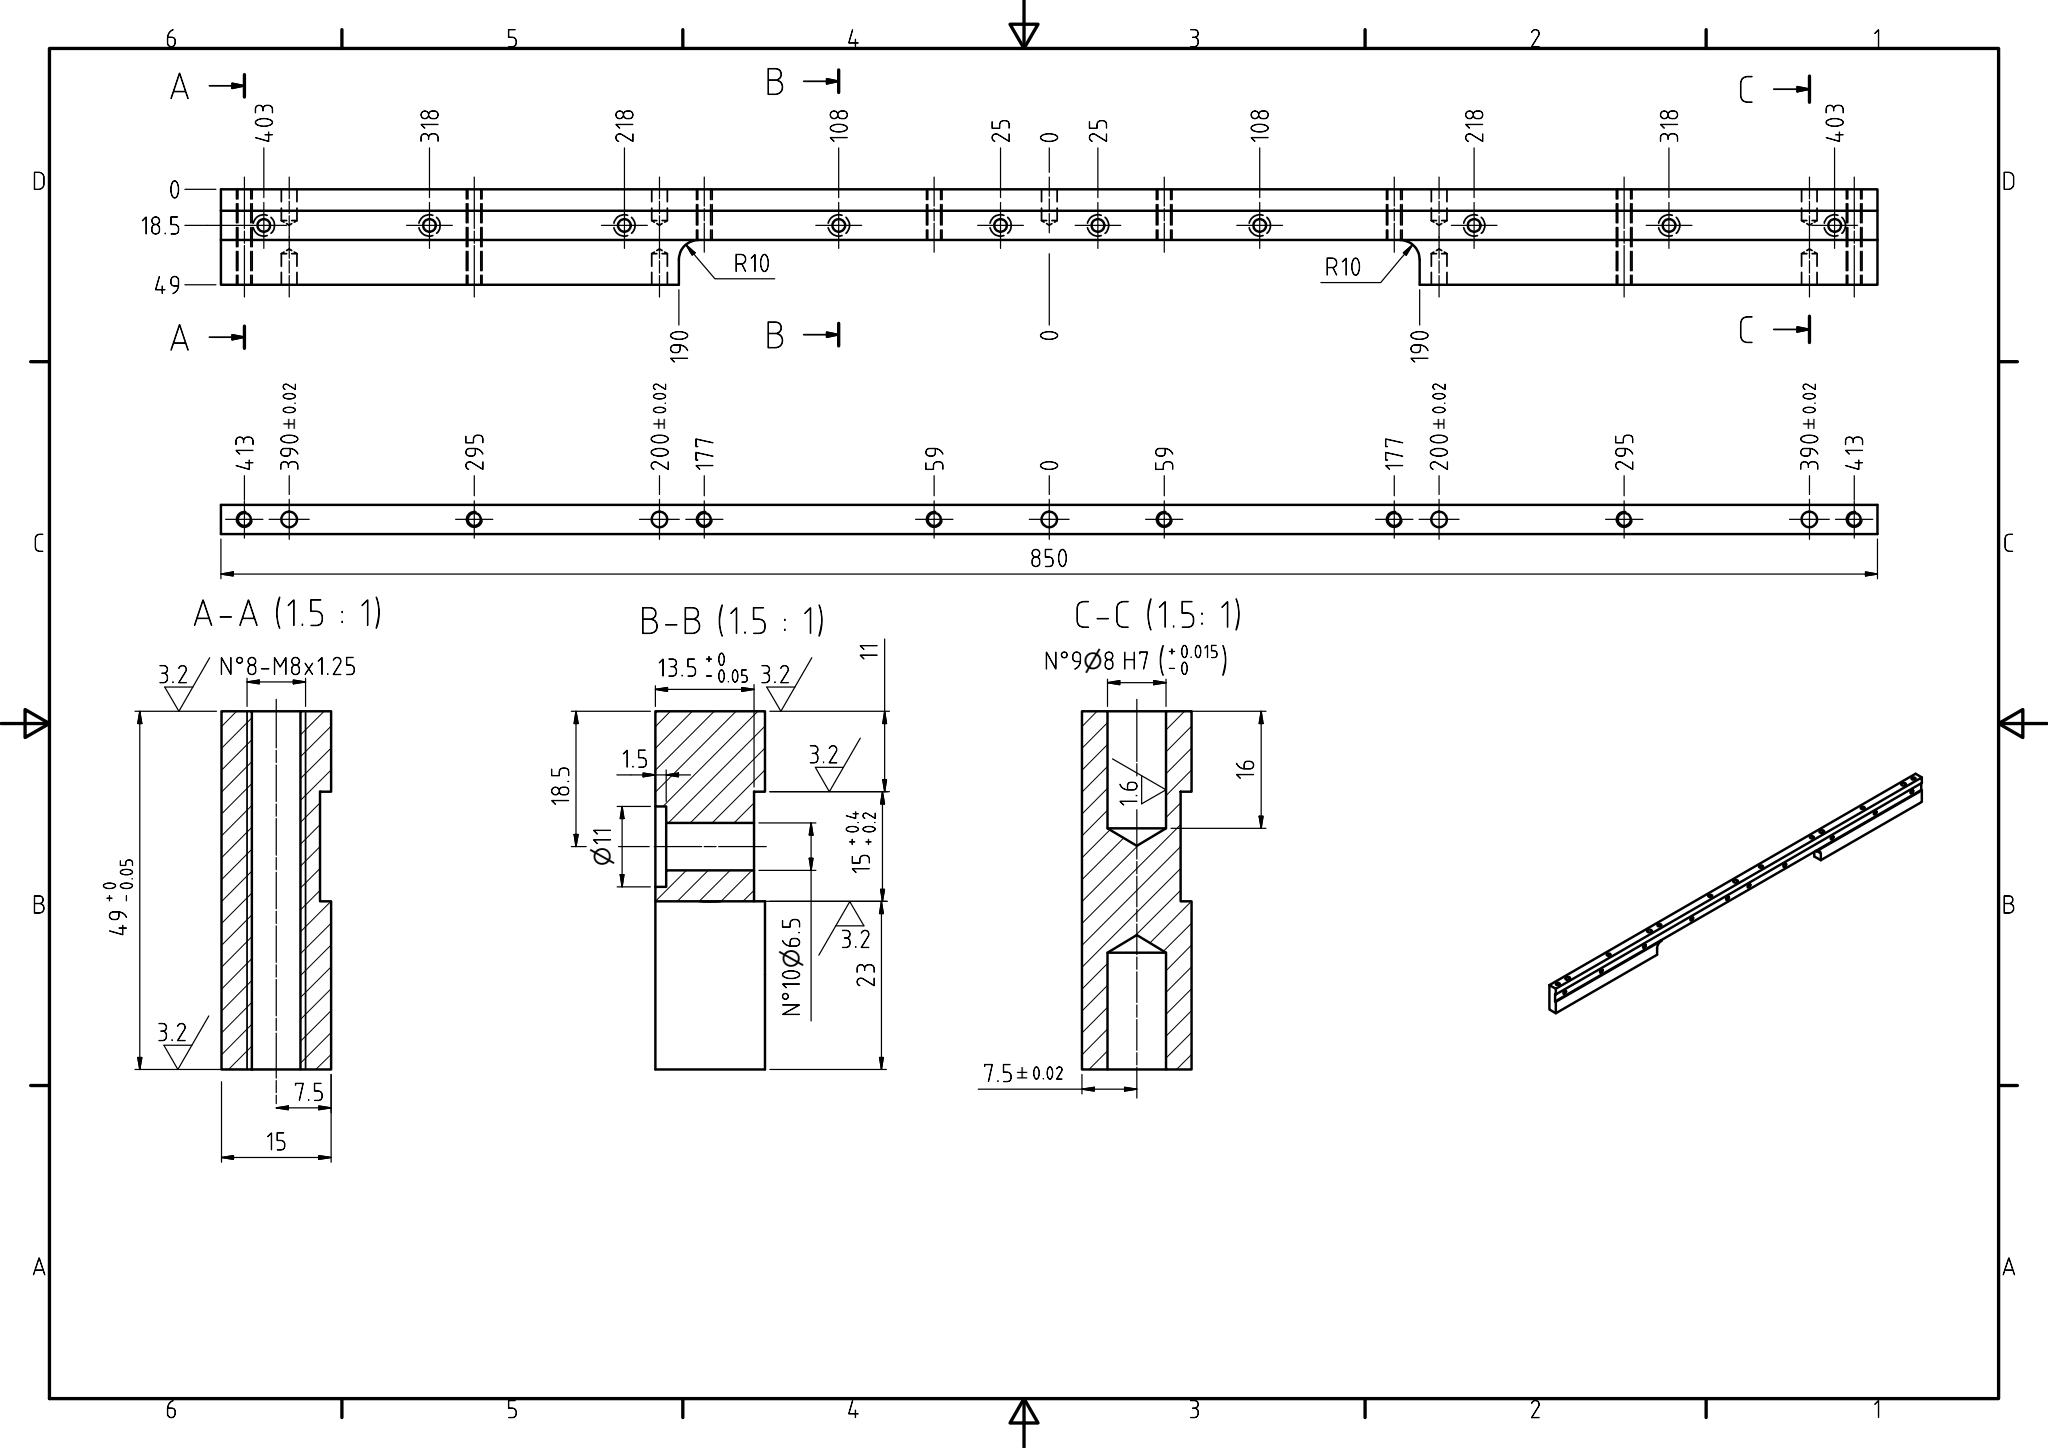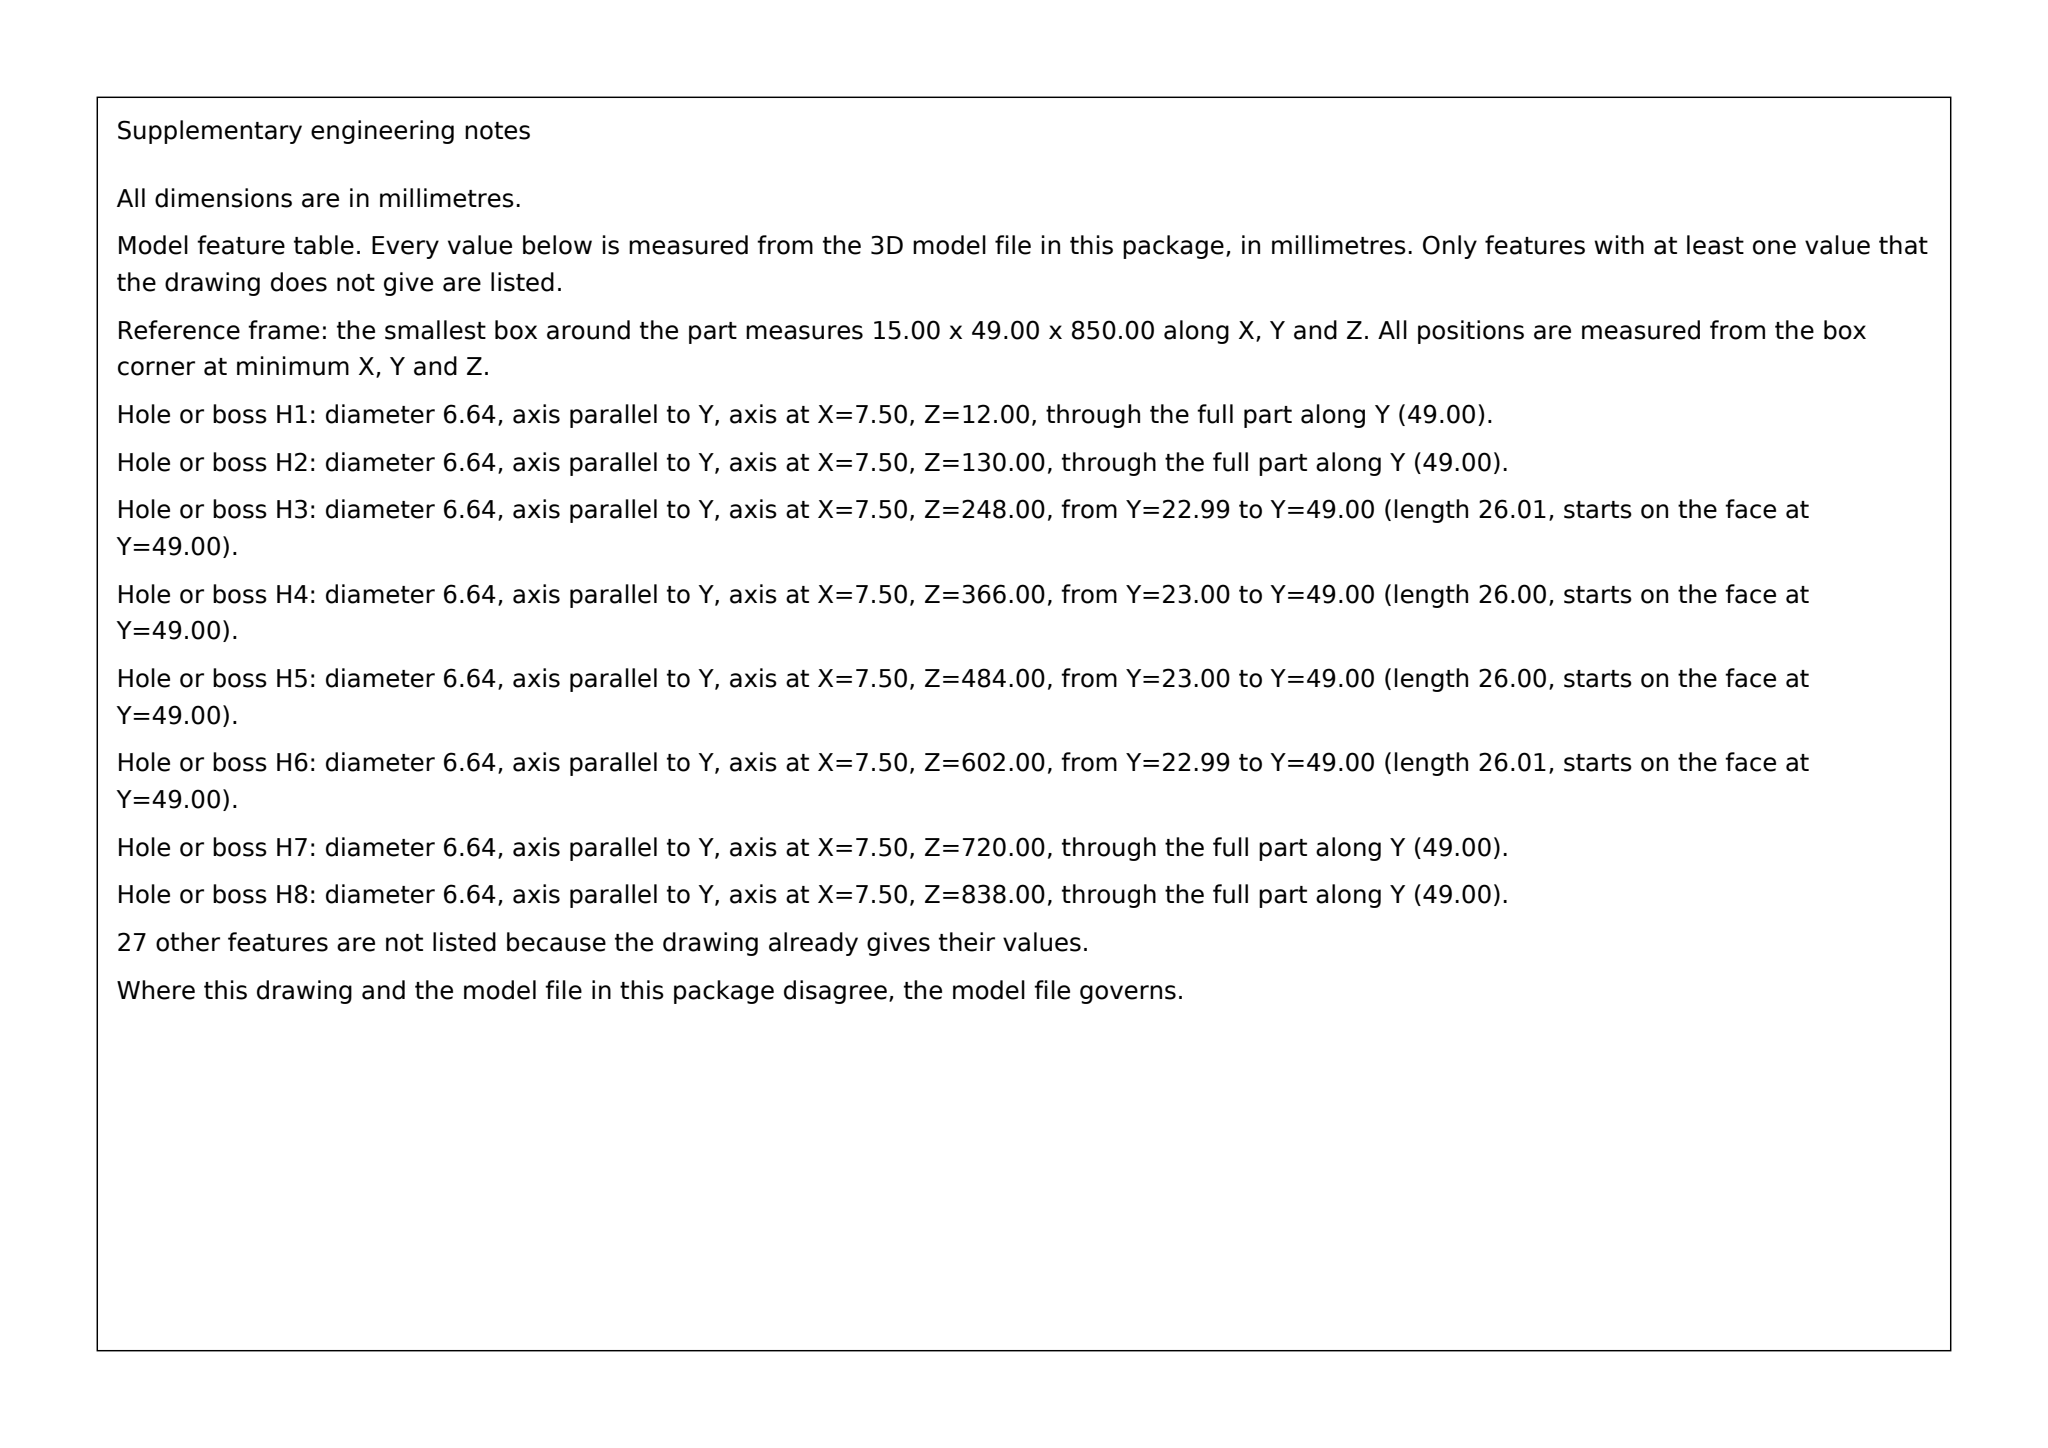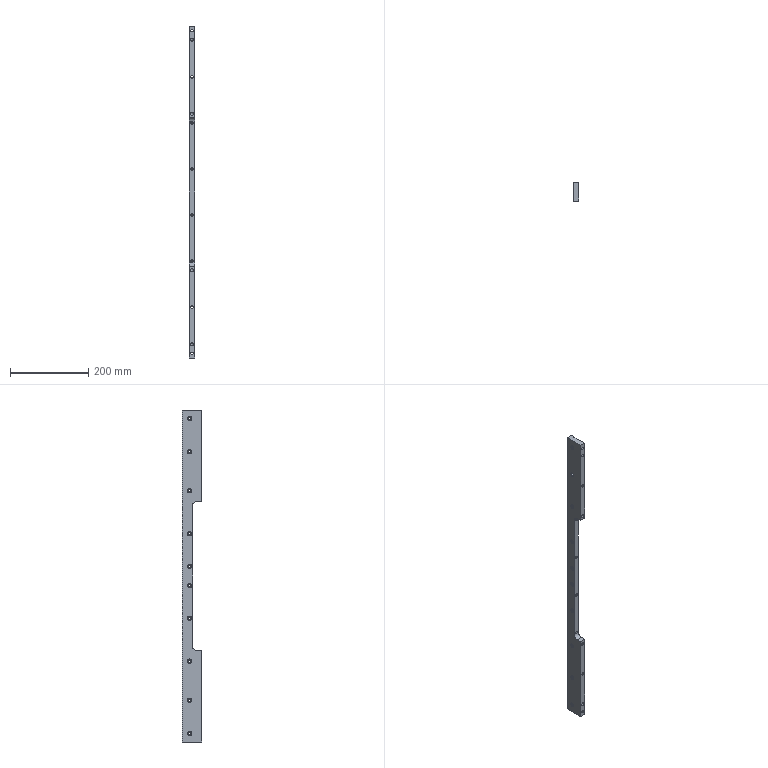Part | SolidWorks | mm | 1 solid | 120 faces | box 15 x 49 x 850 mm | volume 451750 mm3 | cylinder 76 | plane 26 | cone 18 | commonest cylinder face diameters 6.5 x20 11 x20 8 x18 6.647 x16 20 x2